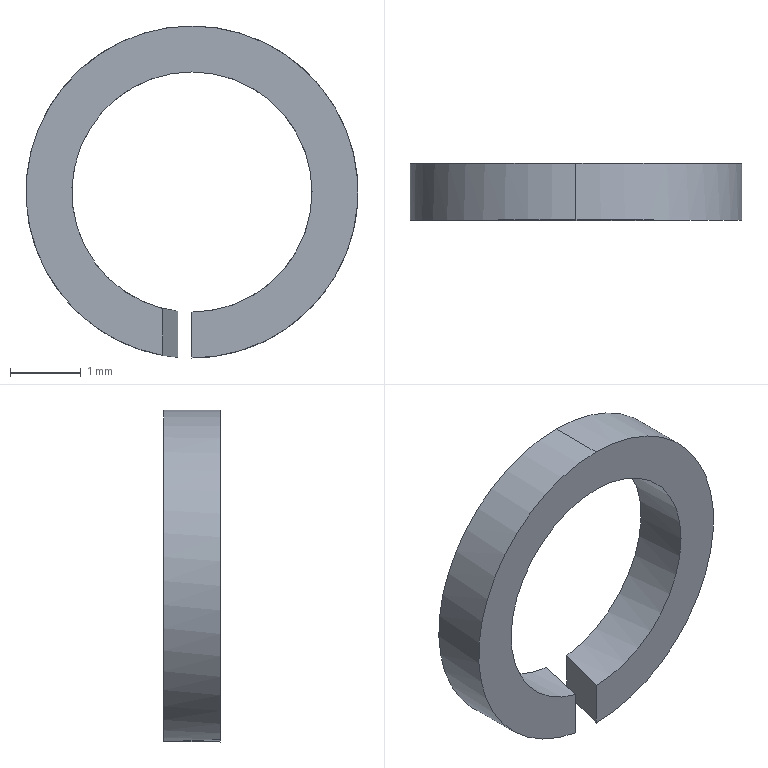Component | SolidWorks | GB 93-87-3-12 | 1 solid | 8 faces | box 4.7 x 0.8 x 4.7 mm | volume 6 mm3 | cylinder 4 | plane 4 | commonest cylinder face diameters 3.4 x2 4.7 x2
build123d program:
from build123d import *

# Parameters (mm, degrees)
SKETCH1_R               = 2.35
SKETCH1_R_2             = 1.7
BOSS_EXTRUDE1_DEPTH     = 0.8
CUT_EXTRUDE1_REACH      = 5.418
CUT_EXTRUDE1_END_RADIUS = 2.35


with BuildPart() as part:
    # Sketch1 → Boss-Extrude1 (new body)
    with BuildSketch(Plane(origin=(0, 0, 0), x_dir=(1, 0, 0), z_dir=(0, 1, 0))):
        with Locations(Location((0, 0, 0), (0, 0, 270))):
            Circle(SKETCH1_R)
        with Locations(Location((0, 0, 0), (0, 0, 270))):
            Circle(SKETCH1_R_2, mode=Mode.SUBTRACT)
    extrude(amount=BOSS_EXTRUDE1_DEPTH)

    # Cut-Extrude1: up to this cylinder (the profile starts inside it)
    cut_extrude1_end = Plane(origin=(0, 0.4, 0), z_dir=(0, -1, 0)) * Cylinder(CUT_EXTRUDE1_END_RADIUS, 16.536, mode=Mode.PRIVATE)
    # Sketch2 → Cut-Extrude1 (cut, up to the surface)
    with BuildSketch(Plane.XY, mode=Mode.PRIVATE) as cut_extrude1_sk1:
        Polygon((0, 0), (-0.2144, 0.8), (0.1998, 0.8), (0.4141, 0), align=None)
    cut_extrude1_tool1 = extrude(cut_extrude1_sk1.sketch, amount=CUT_EXTRUDE1_REACH, mode=Mode.PRIVATE) & cut_extrude1_end
    add(cut_extrude1_tool1.solids().sort_by_distance((0.09988, 0.4, 0))[0], mode=Mode.SUBTRACT)


solid = part.part

# Placed as in the assembly
solid = solid.moved(Location((19.903, 19.517, 28), (-180, 0, 180)))
STEP:
#1=CARTESIAN_POINT('',(0.7757,0.7999,1.036));
#2=VERTEX_POINT('',#1);
#3=CARTESIAN_POINT('',(0.7836,0.7999,1.169));
#4=VERTEX_POINT('',#3);
#5=CARTESIAN_POINT('',(0.7836,0.7999,1.102));
#6=DIRECTION('',(0.,1.,-0.));
#7=DIRECTION('',(0.,0.,-1.));
#8=AXIS2_PLACEMENT_3D('',#5,#6,#7);
#9=CIRCLE('',#8,0.06693);
#10=EDGE_CURVE('',#2,#4,#9,.T.);
#11=ORIENTED_EDGE('',*,*,#10,.T.);
#12=CARTESIAN_POINT('',(0.7836,0.7684,1.169));
#13=VERTEX_POINT('',#12);
#14=CARTESIAN_POINT('',(0.7836,0.7999,1.169));
#15=DIRECTION('',(-0.,-1.,0.));
#16=VECTOR('',#15,39.37);
#17=LINE('',#14,#16);
#18=EDGE_CURVE('',#4,#13,#17,.T.);
#19=ORIENTED_EDGE('',*,*,#18,.T.);
#20=CARTESIAN_POINT('',(0.7673,0.7684,1.037));
#21=VERTEX_POINT('',#20);
#22=CARTESIAN_POINT('',(0.7836,0.7684,1.102));
#23=DIRECTION('',(0.,1.,-0.));
#24=DIRECTION('',(0.,0.,-1.));
#25=AXIS2_PLACEMENT_3D('',#22,#23,#24);
#26=CIRCLE('',#25,0.06693);
#27=EDGE_CURVE('',#21,#13,#26,.T.);
#28=ORIENTED_EDGE('',*,*,#27,.F.);
#29=CARTESIAN_POINT('',(0.7757,0.7999,1.036));
#30=CARTESIAN_POINT('',(0.7729,0.7893,1.036));
#31=CARTESIAN_POINT('',(0.7701,0.7788,1.037));
#32=CARTESIAN_POINT('',(0.7673,0.7684,1.037));
#33=(BOUNDED_CURVE()B_SPLINE_CURVE(3,(#29,#30,#31,#32),.UNSPECIFIED.,.F.,.T.)B_SPLINE_CURVE_WITH_KNOTS((4,4),(4.83,4.958),.UNSPECIFIED.)CURVE()GEOMETRIC_REPRESENTATION_ITEM()RATIONAL_B_SPLINE_CURVE((1.,0.9986,0.9986,1.))REPRESENTATION_ITEM(''));
#34=EDGE_CURVE('',#2,#21,#33,.T.);
#35=ORIENTED_EDGE('',*,*,#34,.F.);
#36=EDGE_LOOP('',(#11,#19,#28,#35));
#37=FACE_OUTER_BOUND('',#36,.T.);
#38=CARTESIAN_POINT('',(0.7836,0.7999,1.102));
#39=DIRECTION('',(-0.,-1.,0.));
#40=DIRECTION('',(0.,0.,1.));
#41=AXIS2_PLACEMENT_3D('',#38,#39,#40);
#42=CYLINDRICAL_SURFACE('',#41,0.06693);
#43=ADVANCED_FACE('',(#37),#42,.F.);
#44=CARTESIAN_POINT('',(0.7836,0.7999,1.195));
#45=VERTEX_POINT('',#44);
#46=CARTESIAN_POINT('',(0.792,0.7999,1.01));
#47=VERTEX_POINT('',#46);
#48=CARTESIAN_POINT('',(0.7836,0.7999,1.102));
#49=DIRECTION('',(0.,1.,-0.));
#50=DIRECTION('',(0.,0.,-1.));
#51=AXIS2_PLACEMENT_3D('',#48,#49,#50);
#52=CIRCLE('',#51,0.09252);
#53=EDGE_CURVE('',#45,#47,#52,.T.);
#54=ORIENTED_EDGE('',*,*,#53,.F.);
#55=CARTESIAN_POINT('',(0.7836,0.7684,1.195));
#56=VERTEX_POINT('',#55);
#57=CARTESIAN_POINT('',(0.7836,0.7999,1.195));
#58=DIRECTION('',(-0.,-1.,0.));
#59=VECTOR('',#58,39.37);
#60=LINE('',#57,#59);
#61=EDGE_CURVE('',#45,#56,#60,.T.);
#62=ORIENTED_EDGE('',*,*,#61,.T.);
#63=CARTESIAN_POINT('',(0.7836,0.7684,1.01));
#64=VERTEX_POINT('',#63);
#65=CARTESIAN_POINT('',(0.7836,0.7684,1.102));
#66=DIRECTION('',(0.,1.,-0.));
#67=DIRECTION('',(0.,0.,-1.));
#68=AXIS2_PLACEMENT_3D('',#65,#66,#67);
#69=CIRCLE('',#68,0.09252);
#70=EDGE_CURVE('',#56,#64,#69,.T.);
#71=ORIENTED_EDGE('',*,*,#70,.T.);
#72=CARTESIAN_POINT('',(0.7836,0.7684,1.01));
#73=CARTESIAN_POINT('',(0.7864,0.7789,1.01));
#74=CARTESIAN_POINT('',(0.7892,0.7894,1.01));
#75=CARTESIAN_POINT('',(0.792,0.7999,1.01));
#76=(BOUNDED_CURVE()B_SPLINE_CURVE(3,(#72,#73,#74,#75),.UNSPECIFIED.,.F.,.F.)B_SPLINE_CURVE_WITH_KNOTS((4,4),(1.571,1.662),.UNSPECIFIED.)CURVE()GEOMETRIC_REPRESENTATION_ITEM()RATIONAL_B_SPLINE_CURVE((1.,0.9993,0.9993,1.))REPRESENTATION_ITEM(''));
#77=EDGE_CURVE('',#64,#47,#76,.T.);
#78=ORIENTED_EDGE('',*,*,#77,.T.);
#79=EDGE_LOOP('',(#54,#62,#71,#78));
#80=FACE_OUTER_BOUND('',#79,.T.);
#81=CARTESIAN_POINT('',(0.7836,0.7999,1.102));
#82=DIRECTION('',(-0.,-1.,0.));
#83=DIRECTION('',(0.,0.,1.));
#84=AXIS2_PLACEMENT_3D('',#81,#82,#83);
#85=CYLINDRICAL_SURFACE('',#84,0.09252);
#86=ADVANCED_FACE('',(#80),#85,.T.);
#87=ORIENTED_EDGE('',*,*,#10,.F.);
#88=CARTESIAN_POINT('',(0.7757,0.7999,1.01));
#89=VERTEX_POINT('',#88);
#90=CARTESIAN_POINT('',(0.7757,0.7999,1.01));
#91=DIRECTION('',(-0.,0.,1.));
#92=VECTOR('',#91,39.37);
#93=LINE('',#90,#92);
#94=EDGE_CURVE('',#89,#2,#93,.T.);
#95=ORIENTED_EDGE('',*,*,#94,.F.);
#96=CARTESIAN_POINT('',(0.7836,0.7999,1.102));
#97=DIRECTION('',(0.,1.,-0.));
#98=DIRECTION('',(0.,0.,-1.));
#99=AXIS2_PLACEMENT_3D('',#96,#97,#98);
#100=CIRCLE('',#99,0.09252);
#101=EDGE_CURVE('',#89,#45,#100,.T.);
#102=ORIENTED_EDGE('',*,*,#101,.T.);
#103=ORIENTED_EDGE('',*,*,#53,.T.);
#104=CARTESIAN_POINT('',(0.792,0.7999,1.036));
#105=VERTEX_POINT('',#104);
#106=CARTESIAN_POINT('',(0.792,0.7999,1.01));
#107=DIRECTION('',(-0.,0.,1.));
#108=VECTOR('',#107,39.37);
#109=LINE('',#106,#108);
#110=EDGE_CURVE('',#47,#105,#109,.T.);
#111=ORIENTED_EDGE('',*,*,#110,.T.);
#112=CARTESIAN_POINT('',(0.7836,0.7999,1.102));
#113=DIRECTION('',(0.,1.,-0.));
#114=DIRECTION('',(0.,0.,-1.));
#115=AXIS2_PLACEMENT_3D('',#112,#113,#114);
#116=CIRCLE('',#115,0.06693);
#117=EDGE_CURVE('',#4,#105,#116,.T.);
#118=ORIENTED_EDGE('',*,*,#117,.F.);
#119=EDGE_LOOP('',(#87,#95,#102,#103,#111,#118));
#120=FACE_OUTER_BOUND('',#119,.T.);
#121=CARTESIAN_POINT('',(0.7836,0.7999,1.102));
#122=DIRECTION('',(0.,1.,-0.));
#123=DIRECTION('',(0.,-0.,-1.));
#124=AXIS2_PLACEMENT_3D('',#121,#122,#123);
#125=PLANE('',#124);
#126=ADVANCED_FACE('',(#120),#125,.T.);
#127=CARTESIAN_POINT('',(0.7673,0.7684,1.011));
#128=VERTEX_POINT('',#127);
#129=CARTESIAN_POINT('',(0.7673,0.7684,1.01));
#130=DIRECTION('',(-0.,0.,1.));
#131=VECTOR('',#130,39.37);
#132=LINE('',#129,#131);
#133=EDGE_CURVE('',#128,#21,#132,.T.);
#134=ORIENTED_EDGE('',*,*,#133,.T.);
#135=ORIENTED_EDGE('',*,*,#27,.T.);
#136=CARTESIAN_POINT('',(0.7836,0.7684,1.035));
#137=VERTEX_POINT('',#136);
#138=CARTESIAN_POINT('',(0.7836,0.7684,1.102));
#139=DIRECTION('',(0.,1.,-0.));
#140=DIRECTION('',(0.,0.,-1.));
#141=AXIS2_PLACEMENT_3D('',#138,#139,#140);
#142=CIRCLE('',#141,0.06693);
#143=EDGE_CURVE('',#13,#137,#142,.T.);
#144=ORIENTED_EDGE('',*,*,#143,.T.);
#145=CARTESIAN_POINT('',(0.7836,0.7684,1.01));
#146=DIRECTION('',(-0.,0.,1.));
#147=VECTOR('',#146,39.37);
#148=LINE('',#145,#147);
#149=EDGE_CURVE('',#64,#137,#148,.T.);
#150=ORIENTED_EDGE('',*,*,#149,.F.);
#151=ORIENTED_EDGE('',*,*,#70,.F.);
#152=CARTESIAN_POINT('',(0.7836,0.7684,1.102));
#153=DIRECTION('',(0.,1.,-0.));
#154=DIRECTION('',(0.,0.,-1.));
#155=AXIS2_PLACEMENT_3D('',#152,#153,#154);
#156=CIRCLE('',#155,0.09252);
#157=EDGE_CURVE('',#128,#56,#156,.T.);
#158=ORIENTED_EDGE('',*,*,#157,.F.);
#159=EDGE_LOOP('',(#134,#135,#144,#150,#151,#158));
#160=FACE_OUTER_BOUND('',#159,.T.);
#161=CARTESIAN_POINT('',(0.7836,0.7684,1.102));
#162=DIRECTION('',(0.,1.,-0.));
#163=DIRECTION('',(0.,-0.,-1.));
#164=AXIS2_PLACEMENT_3D('',#161,#162,#163);
#165=PLANE('',#164);
#166=ADVANCED_FACE('',(#160),#165,.F.);
#167=ORIENTED_EDGE('',*,*,#61,.F.);
#168=ORIENTED_EDGE('',*,*,#101,.F.);
#169=CARTESIAN_POINT('',(0.7757,0.7999,1.01));
#170=CARTESIAN_POINT('',(0.7729,0.7893,1.01));
#171=CARTESIAN_POINT('',(0.7701,0.7788,1.011));
#172=CARTESIAN_POINT('',(0.7673,0.7684,1.011));
#173=(BOUNDED_CURVE()B_SPLINE_CURVE(3,(#169,#170,#171,#172),.UNSPECIFIED.,.F.,.T.)B_SPLINE_CURVE_WITH_KNOTS((4,4),(4.797,4.89),.UNSPECIFIED.)CURVE()GEOMETRIC_REPRESENTATION_ITEM()RATIONAL_B_SPLINE_CURVE((1.,0.9993,0.9993,1.))REPRESENTATION_ITEM(''));
#174=EDGE_CURVE('',#89,#128,#173,.T.);
#175=ORIENTED_EDGE('',*,*,#174,.T.);
#176=ORIENTED_EDGE('',*,*,#157,.T.);
#177=EDGE_LOOP('',(#167,#168,#175,#176));
#178=FACE_OUTER_BOUND('',#177,.T.);
#179=CARTESIAN_POINT('',(0.7836,0.7999,1.102));
#180=DIRECTION('',(-0.,-1.,0.));
#181=DIRECTION('',(0.,0.,1.));
#182=AXIS2_PLACEMENT_3D('',#179,#180,#181);
#183=CYLINDRICAL_SURFACE('',#182,0.09252);
#184=ADVANCED_FACE('',(#178),#183,.T.);
#185=ORIENTED_EDGE('',*,*,#18,.F.);
#186=ORIENTED_EDGE('',*,*,#117,.T.);
#187=CARTESIAN_POINT('',(0.7836,0.7684,1.035));
#188=CARTESIAN_POINT('',(0.7864,0.7789,1.035));
#189=CARTESIAN_POINT('',(0.7892,0.7894,1.036));
#190=CARTESIAN_POINT('',(0.792,0.7999,1.036));
#191=(BOUNDED_CURVE()B_SPLINE_CURVE(3,(#187,#188,#189,#190),.UNSPECIFIED.,.F.,.T.)B_SPLINE_CURVE_WITH_KNOTS((4,4),(1.571,1.697),.UNSPECIFIED.)CURVE()GEOMETRIC_REPRESENTATION_ITEM()RATIONAL_B_SPLINE_CURVE((1.,0.9987,0.9987,1.))REPRESENTATION_ITEM(''));
#192=EDGE_CURVE('',#137,#105,#191,.T.);
#193=ORIENTED_EDGE('',*,*,#192,.F.);
#194=ORIENTED_EDGE('',*,*,#143,.F.);
#195=EDGE_LOOP('',(#185,#186,#193,#194));
#196=FACE_OUTER_BOUND('',#195,.T.);
#197=CARTESIAN_POINT('',(0.7836,0.7999,1.102));
#198=DIRECTION('',(-0.,-1.,0.));
#199=DIRECTION('',(0.,0.,1.));
#200=AXIS2_PLACEMENT_3D('',#197,#198,#199);
#201=CYLINDRICAL_SURFACE('',#200,0.06693);
#202=ADVANCED_FACE('',(#196),#201,.F.);
#203=ORIENTED_EDGE('',*,*,#149,.T.);
#204=ORIENTED_EDGE('',*,*,#192,.T.);
#205=ORIENTED_EDGE('',*,*,#110,.F.);
#206=ORIENTED_EDGE('',*,*,#77,.F.);
#207=EDGE_LOOP('',(#203,#204,#205,#206));
#208=FACE_OUTER_BOUND('',#207,.T.);
#209=CARTESIAN_POINT('',(0.7836,0.7684,1.01));
#210=DIRECTION('',(-0.9659,0.2588,-0.));
#211=DIRECTION('',(0.2588,0.9659,0.));
#212=AXIS2_PLACEMENT_3D('',#209,#210,#211);
#213=PLANE('',#212);
#214=ADVANCED_FACE('',(#208),#213,.T.);
#215=ORIENTED_EDGE('',*,*,#94,.T.);
#216=ORIENTED_EDGE('',*,*,#34,.T.);
#217=ORIENTED_EDGE('',*,*,#133,.F.);
#218=ORIENTED_EDGE('',*,*,#174,.F.);
#219=EDGE_LOOP('',(#215,#216,#217,#218));
#220=FACE_OUTER_BOUND('',#219,.T.);
#221=CARTESIAN_POINT('',(0.7673,0.7684,1.01));
#222=DIRECTION('',(0.9659,-0.2588,0.));
#223=DIRECTION('',(-0.2588,-0.9659,-0.));
#224=AXIS2_PLACEMENT_3D('',#221,#222,#223);
#225=PLANE('',#224);
#226=ADVANCED_FACE('',(#220),#225,.T.);
#227=CLOSED_SHELL('',(#43,#86,#126,#166,#184,#202,#214,#226));
#228=MANIFOLD_SOLID_BREP('',#227);
#229=CARTESIAN_POINT('',(0.,0.,0.));
#230=DIRECTION('',(0.,0.,1.));
#231=DIRECTION('',(1.,0.,0.));
#232=AXIS2_PLACEMENT_3D('',#229,#230,#231);
#233=(LENGTH_UNIT()NAMED_UNIT(*)SI_UNIT($,.METRE.));
#234=LENGTH_MEASURE_WITH_UNIT(LENGTH_MEASURE(0.0254),#233);
#235=DIMENSIONAL_EXPONENTS(1.,0.,0.,0.,0.,0.,0.);
#236=(CONVERSION_BASED_UNIT('',#234)LENGTH_UNIT()NAMED_UNIT(#235));
#237=UNCERTAINTY_MEASURE_WITH_UNIT(LENGTH_MEASURE(0.00001),#236,'','');
#238=(NAMED_UNIT(*)PLANE_ANGLE_UNIT()SI_UNIT($,.RADIAN.));
#239=(NAMED_UNIT(*)SI_UNIT($,.STERADIAN.)SOLID_ANGLE_UNIT());
#240=(GEOMETRIC_REPRESENTATION_CONTEXT(3)GLOBAL_UNCERTAINTY_ASSIGNED_CONTEXT((#237))GLOBAL_UNIT_ASSIGNED_CONTEXT((#236,#238,#239))REPRESENTATION_CONTEXT('',''));
#241=ADVANCED_BREP_SHAPE_REPRESENTATION('',(#228,#232),#240);
#242=COLOUR_RGB('',0.7922,0.8196,0.9333);
#243=FILL_AREA_STYLE_COLOUR('',#242);
#244=FILL_AREA_STYLE('',(#243));
#245=SURFACE_STYLE_FILL_AREA(#244);
#246=SURFACE_SIDE_STYLE('',(#245));
#247=SURFACE_STYLE_USAGE(.BOTH.,#246);
#248=PRESENTATION_STYLE_ASSIGNMENT((#247));
#249=STYLED_ITEM('',(#248),#228);
#250=(LENGTH_UNIT()NAMED_UNIT(*)SI_UNIT($,.METRE.));
#251=LENGTH_MEASURE_WITH_UNIT(LENGTH_MEASURE(0.0254),#250);
#252=DIMENSIONAL_EXPONENTS(1.,0.,0.,0.,0.,0.,0.);
#253=(CONVERSION_BASED_UNIT('',#251)LENGTH_UNIT()NAMED_UNIT(#252));
#254=UNCERTAINTY_MEASURE_WITH_UNIT(LENGTH_MEASURE(0.00001),#253,'','');
#255=(NAMED_UNIT(*)PLANE_ANGLE_UNIT()SI_UNIT($,.RADIAN.));
#256=(NAMED_UNIT(*)SI_UNIT($,.STERADIAN.)SOLID_ANGLE_UNIT());
#257=(GEOMETRIC_REPRESENTATION_CONTEXT(3)GLOBAL_UNCERTAINTY_ASSIGNED_CONTEXT((#254))GLOBAL_UNIT_ASSIGNED_CONTEXT((#253,#255,#256))REPRESENTATION_CONTEXT('',''));
#258=MECHANICAL_DESIGN_GEOMETRIC_PRESENTATION_REPRESENTATION('',(#249),#257);
#259=PRESENTATION_LAYER_ASSIGNMENT('','',(#249));